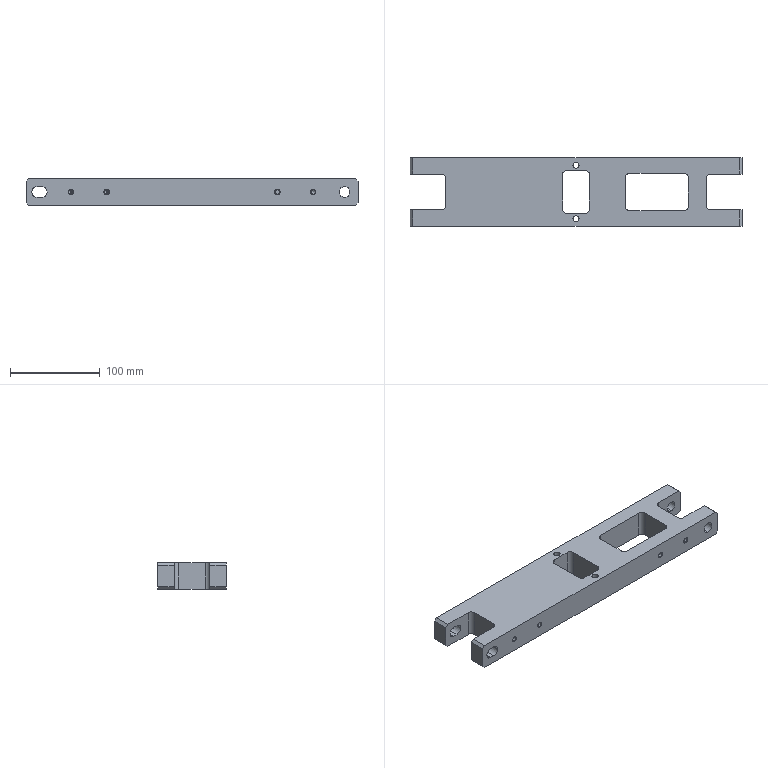Component | SolidWorks | DirectPressureVerticalSeal-1_MainArm-1 | 1 solid | 122 faces | volume 599880 mm3 | cylinder 47 | cone 40 | plane 35 | commonest cylinder face diameters 5 x16 10 x13 12 x10 8.5 x4 6.8 x4